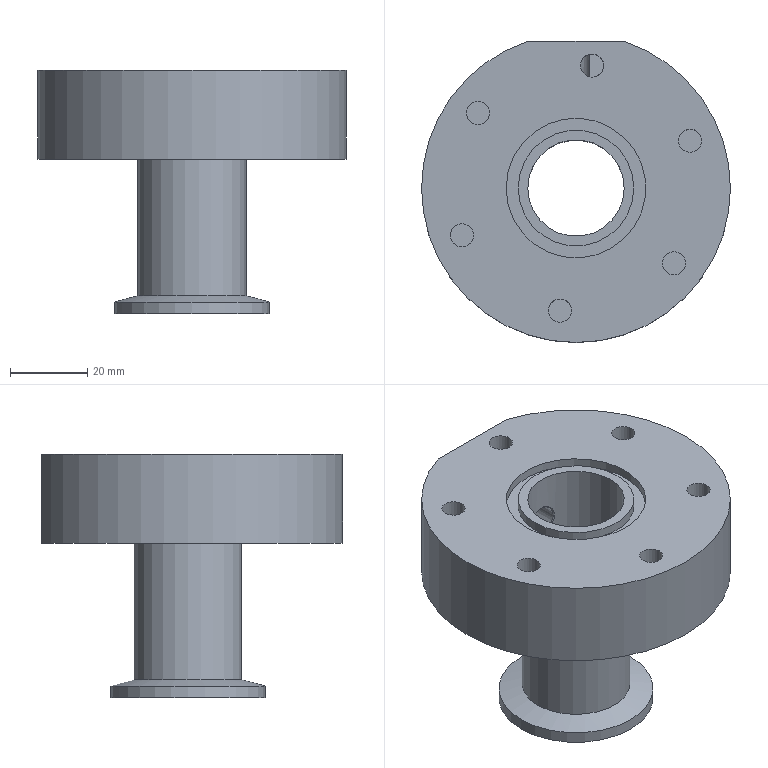Component | NX | CH3404_1-4 | 1 solid | 29 faces | volume 106938 mm3 | cylinder 14 | plane 13 | cone 1 | spline 1 | commonest cylinder face diameters 6 x6 80 x1 7.5 x1 28 x1 40 x1 26.2 x1 25 x1 30 x1